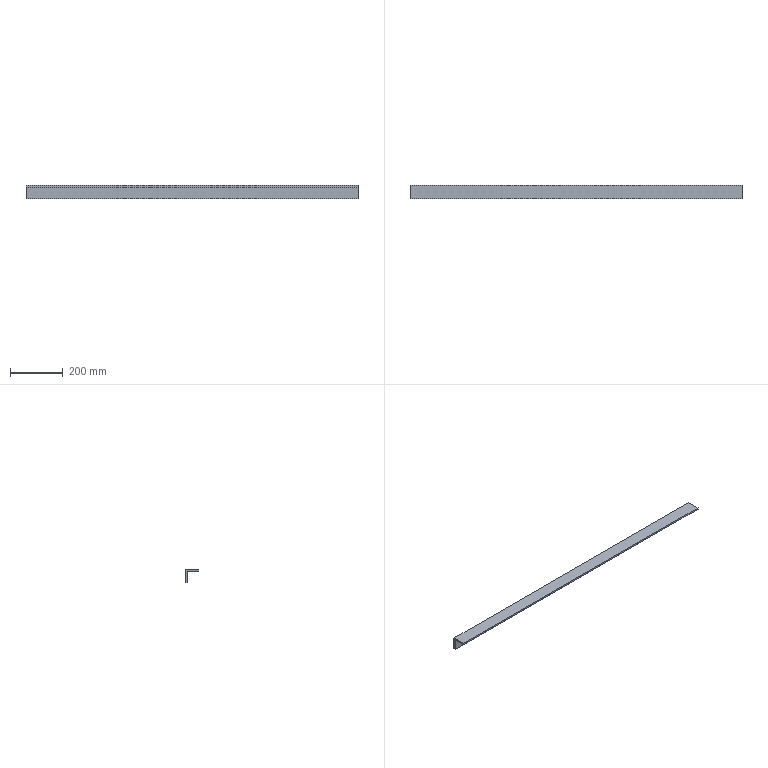Component | NX | LENGTH_CORNER_PROTECTOR_2 | 1 solid | 8 faces | box 1262 x 50 x 50 mm | volume 711768 mm3 | plane 8
STEP:
#1=CARTESIAN_POINT('',(0.,0.,0.));
#2=DIRECTION('',(0.,0.,1.));
#3=DIRECTION('',(1.,0.,0.));
#4=AXIS2_PLACEMENT_3D('',#1,#2,#3);
#5=CARTESIAN_POINT('',(633.5,527.,931.));
#6=VERTEX_POINT('',#5);
#7=CARTESIAN_POINT('',(633.5,527.,981.));
#8=VERTEX_POINT('',#7);
#9=CARTESIAN_POINT('',(633.5,527.,0.));
#10=DIRECTION('',(0.,-0.,1.));
#11=VECTOR('',#10,1.);
#12=LINE('',#9,#11);
#13=CARTESIAN_POINT('',(633.5,-1095.,990.));
#14=DIRECTION('',(-1.,0.,0.));
#15=DIRECTION('',(0.,0.,1.));
#16=AXIS2_PLACEMENT_3D('',#13,#14,#15);
#17=PLANE('',#16);
#18=CARTESIAN_POINT('',(-990.,1622.));
#19=DIRECTION('',(1.,-0.));
#20=VECTOR('',#19,1.);
#21=LINE('',#18,#20);
#22=(GEOMETRIC_REPRESENTATION_CONTEXT(2)PARAMETRIC_REPRESENTATION_CONTEXT()REPRESENTATION_CONTEXT('',''));
#23=DEFINITIONAL_REPRESENTATION('',(#21),#22);
#24=PCURVE('',#17,#23);
#25=CARTESIAN_POINT('',(-628.5,527.,0.));
#26=DIRECTION('',(-0.,1.,0.));
#27=DIRECTION('',(-1.,-0.,0.));
#28=AXIS2_PLACEMENT_3D('',#25,#26,#27);
#29=PLANE('',#28);
#30=CARTESIAN_POINT('',(-1262.,0.));
#31=DIRECTION('',(0.,1.));
#32=VECTOR('',#31,1.);
#33=LINE('',#30,#32);
#34=(GEOMETRIC_REPRESENTATION_CONTEXT(2)PARAMETRIC_REPRESENTATION_CONTEXT()REPRESENTATION_CONTEXT('',''));
#35=DEFINITIONAL_REPRESENTATION('',(#33),#34);
#36=PCURVE('',#29,#35);
#37=SURFACE_CURVE('',#12,(#24,#36),.PCURVE_S1.);
#38=EDGE_CURVE('',#6,#8,#37,.T.);
#39=ORIENTED_EDGE('',*,*,#38,.T.);
#40=CARTESIAN_POINT('',(633.5,477.,981.));
#41=VERTEX_POINT('',#40);
#42=CARTESIAN_POINT('',(633.5,521.,981.));
#43=DIRECTION('',(0.,-1.,0.));
#44=VECTOR('',#43,1.);
#45=LINE('',#42,#44);
#46=CARTESIAN_POINT('',(-9.,1616.));
#47=DIRECTION('',(0.,-1.));
#48=VECTOR('',#47,1.);
#49=LINE('',#46,#48);
#50=(GEOMETRIC_REPRESENTATION_CONTEXT(2)PARAMETRIC_REPRESENTATION_CONTEXT()REPRESENTATION_CONTEXT('',''));
#51=DEFINITIONAL_REPRESENTATION('',(#49),#50);
#52=PCURVE('',#17,#51);
#53=CARTESIAN_POINT('',(-628.5,521.,981.));
#54=DIRECTION('',(0.,0.,1.));
#55=DIRECTION('',(0.7071,0.7071,0.));
#56=AXIS2_PLACEMENT_3D('',#53,#54,#55);
#57=PLANE('',#56);
#58=CARTESIAN_POINT('',(892.369,-892.369));
#59=DIRECTION('',(-0.7071,-0.7071));
#60=VECTOR('',#59,1.);
#61=LINE('',#58,#60);
#62=(GEOMETRIC_REPRESENTATION_CONTEXT(2)PARAMETRIC_REPRESENTATION_CONTEXT()REPRESENTATION_CONTEXT('',''));
#63=DEFINITIONAL_REPRESENTATION('',(#61),#62);
#64=PCURVE('',#57,#63);
#65=SURFACE_CURVE('',#45,(#52,#64),.PCURVE_S1.);
#66=EDGE_CURVE('',#8,#41,#65,.T.);
#67=ORIENTED_EDGE('',*,*,#66,.T.);
#68=CARTESIAN_POINT('',(633.5,477.,975.));
#69=VERTEX_POINT('',#68);
#70=CARTESIAN_POINT('',(633.5,477.,975.));
#71=DIRECTION('',(0.,0.,-1.));
#72=VECTOR('',#71,1.);
#73=LINE('',#70,#72);
#74=CARTESIAN_POINT('',(-15.,1572.));
#75=DIRECTION('',(-1.,0.));
#76=VECTOR('',#75,1.);
#77=LINE('',#74,#76);
#78=(GEOMETRIC_REPRESENTATION_CONTEXT(2)PARAMETRIC_REPRESENTATION_CONTEXT()REPRESENTATION_CONTEXT('',''));
#79=DEFINITIONAL_REPRESENTATION('',(#77),#78);
#80=PCURVE('',#17,#79);
#81=CARTESIAN_POINT('',(-628.5,477.,975.));
#82=DIRECTION('',(0.,-1.,0.));
#83=DIRECTION('',(1.,0.,0.));
#84=AXIS2_PLACEMENT_3D('',#81,#82,#83);
#85=PLANE('',#84);
#86=CARTESIAN_POINT('',(1262.,0.));
#87=DIRECTION('',(0.,-1.));
#88=VECTOR('',#87,1.);
#89=LINE('',#86,#88);
#90=(GEOMETRIC_REPRESENTATION_CONTEXT(2)PARAMETRIC_REPRESENTATION_CONTEXT()REPRESENTATION_CONTEXT('',''));
#91=DEFINITIONAL_REPRESENTATION('',(#89),#90);
#92=PCURVE('',#85,#91);
#93=SURFACE_CURVE('',#73,(#80,#92),.PCURVE_S1.);
#94=EDGE_CURVE('',#41,#69,#93,.T.);
#95=ORIENTED_EDGE('',*,*,#94,.T.);
#96=CARTESIAN_POINT('',(633.5,521.,975.));
#97=VERTEX_POINT('',#96);
#98=CARTESIAN_POINT('',(633.5,521.,975.));
#99=DIRECTION('',(0.,-1.,0.));
#100=VECTOR('',#99,1.);
#101=LINE('',#98,#100);
#102=CARTESIAN_POINT('',(-15.,1616.));
#103=DIRECTION('',(0.,-1.));
#104=VECTOR('',#103,1.);
#105=LINE('',#102,#104);
#106=(GEOMETRIC_REPRESENTATION_CONTEXT(2)PARAMETRIC_REPRESENTATION_CONTEXT()REPRESENTATION_CONTEXT('',''));
#107=DEFINITIONAL_REPRESENTATION('',(#105),#106);
#108=PCURVE('',#17,#107);
#109=CARTESIAN_POINT('',(-628.5,521.,975.));
#110=DIRECTION('',(0.,0.,1.));
#111=DIRECTION('',(0.7071,0.7071,0.));
#112=AXIS2_PLACEMENT_3D('',#109,#110,#111);
#113=PLANE('',#112);
#114=CARTESIAN_POINT('',(892.369,-892.369));
#115=DIRECTION('',(-0.7071,-0.7071));
#116=VECTOR('',#115,1.);
#117=LINE('',#114,#116);
#118=(GEOMETRIC_REPRESENTATION_CONTEXT(2)PARAMETRIC_REPRESENTATION_CONTEXT()REPRESENTATION_CONTEXT('',''));
#119=DEFINITIONAL_REPRESENTATION('',(#117),#118);
#120=PCURVE('',#113,#119);
#121=SURFACE_CURVE('',#101,(#108,#120),.PCURVE_S1.);
#122=EDGE_CURVE('',#97,#69,#121,.T.);
#123=ORIENTED_EDGE('',*,*,#122,.F.);
#124=CARTESIAN_POINT('',(633.5,521.,931.));
#125=VERTEX_POINT('',#124);
#126=CARTESIAN_POINT('',(633.5,521.,0.));
#127=DIRECTION('',(0.,-0.,1.));
#128=VECTOR('',#127,1.);
#129=LINE('',#126,#128);
#130=CARTESIAN_POINT('',(-990.,1616.));
#131=DIRECTION('',(1.,-0.));
#132=VECTOR('',#131,1.);
#133=LINE('',#130,#132);
#134=(GEOMETRIC_REPRESENTATION_CONTEXT(2)PARAMETRIC_REPRESENTATION_CONTEXT()REPRESENTATION_CONTEXT('',''));
#135=DEFINITIONAL_REPRESENTATION('',(#133),#134);
#136=PCURVE('',#17,#135);
#137=CARTESIAN_POINT('',(-628.5,521.,0.));
#138=DIRECTION('',(-0.,1.,0.));
#139=DIRECTION('',(-1.,-0.,0.));
#140=AXIS2_PLACEMENT_3D('',#137,#138,#139);
#141=PLANE('',#140);
#142=CARTESIAN_POINT('',(-1262.,0.));
#143=DIRECTION('',(0.,1.));
#144=VECTOR('',#143,1.);
#145=LINE('',#142,#144);
#146=(GEOMETRIC_REPRESENTATION_CONTEXT(2)PARAMETRIC_REPRESENTATION_CONTEXT()REPRESENTATION_CONTEXT('',''));
#147=DEFINITIONAL_REPRESENTATION('',(#145),#146);
#148=PCURVE('',#141,#147);
#149=SURFACE_CURVE('',#129,(#136,#148),.PCURVE_S1.);
#150=EDGE_CURVE('',#125,#97,#149,.T.);
#151=ORIENTED_EDGE('',*,*,#150,.F.);
#152=CARTESIAN_POINT('',(633.5,521.,931.));
#153=DIRECTION('',(0.,1.,0.));
#154=VECTOR('',#153,1.);
#155=LINE('',#152,#154);
#156=CARTESIAN_POINT('',(-59.,1616.));
#157=DIRECTION('',(0.,1.));
#158=VECTOR('',#157,1.);
#159=LINE('',#156,#158);
#160=(GEOMETRIC_REPRESENTATION_CONTEXT(2)PARAMETRIC_REPRESENTATION_CONTEXT()REPRESENTATION_CONTEXT('',''));
#161=DEFINITIONAL_REPRESENTATION('',(#159),#160);
#162=PCURVE('',#17,#161);
#163=CARTESIAN_POINT('',(-628.5,521.,931.));
#164=DIRECTION('',(0.,-0.,1.));
#165=DIRECTION('',(1.,0.,0.));
#166=AXIS2_PLACEMENT_3D('',#163,#164,#165);
#167=PLANE('',#166);
#168=CARTESIAN_POINT('',(1262.,-0.));
#169=DIRECTION('',(0.,1.));
#170=VECTOR('',#169,1.);
#171=LINE('',#168,#170);
#172=(GEOMETRIC_REPRESENTATION_CONTEXT(2)PARAMETRIC_REPRESENTATION_CONTEXT()REPRESENTATION_CONTEXT('',''));
#173=DEFINITIONAL_REPRESENTATION('',(#171),#172);
#174=PCURVE('',#167,#173);
#175=SURFACE_CURVE('',#155,(#162,#174),.PCURVE_S1.);
#176=EDGE_CURVE('',#125,#6,#175,.T.);
#177=ORIENTED_EDGE('',*,*,#176,.T.);
#178=EDGE_LOOP('',(#39,#67,#95,#123,#151,#177));
#179=FACE_BOUND('',#178,.T.);
#180=ADVANCED_FACE('',(#179),#17,.F.);
#181=ORIENTED_EDGE('',*,*,#176,.F.);
#182=CARTESIAN_POINT('',(-628.5,521.,931.));
#183=VERTEX_POINT('',#182);
#184=CARTESIAN_POINT('',(-628.5,521.,931.));
#185=DIRECTION('',(1.,0.,0.));
#186=VECTOR('',#185,1.);
#187=LINE('',#184,#186);
#188=CARTESIAN_POINT('',(0.,0.));
#189=DIRECTION('',(1.,0.));
#190=VECTOR('',#189,1.);
#191=LINE('',#188,#190);
#192=(GEOMETRIC_REPRESENTATION_CONTEXT(2)PARAMETRIC_REPRESENTATION_CONTEXT()REPRESENTATION_CONTEXT('',''));
#193=DEFINITIONAL_REPRESENTATION('',(#191),#192);
#194=PCURVE('',#167,#193);
#195=CARTESIAN_POINT('',(0.,931.));
#196=DIRECTION('',(-1.,0.));
#197=VECTOR('',#196,1.);
#198=LINE('',#195,#197);
#199=(GEOMETRIC_REPRESENTATION_CONTEXT(2)PARAMETRIC_REPRESENTATION_CONTEXT()REPRESENTATION_CONTEXT('',''));
#200=DEFINITIONAL_REPRESENTATION('',(#198),#199);
#201=PCURVE('',#141,#200);
#202=SURFACE_CURVE('',#187,(#194,#201),.PCURVE_S1.);
#203=EDGE_CURVE('',#183,#125,#202,.T.);
#204=ORIENTED_EDGE('',*,*,#203,.F.);
#205=CARTESIAN_POINT('',(-628.5,527.,931.));
#206=VERTEX_POINT('',#205);
#207=CARTESIAN_POINT('',(-628.5,521.,931.));
#208=DIRECTION('',(-0.,1.,0.));
#209=VECTOR('',#208,1.);
#210=LINE('',#207,#209);
#211=CARTESIAN_POINT('',(0.,0.));
#212=DIRECTION('',(0.,1.));
#213=VECTOR('',#212,1.);
#214=LINE('',#211,#213);
#215=(GEOMETRIC_REPRESENTATION_CONTEXT(2)PARAMETRIC_REPRESENTATION_CONTEXT()REPRESENTATION_CONTEXT('',''));
#216=DEFINITIONAL_REPRESENTATION('',(#214),#215);
#217=PCURVE('',#167,#216);
#218=CARTESIAN_POINT('',(-628.5,521.,975.));
#219=DIRECTION('',(-1.,-0.,0.));
#220=DIRECTION('',(0.,-1.,0.));
#221=AXIS2_PLACEMENT_3D('',#218,#219,#220);
#222=PLANE('',#221);
#223=CARTESIAN_POINT('',(0.,-44.));
#224=DIRECTION('',(-1.,0.));
#225=VECTOR('',#224,1.);
#226=LINE('',#223,#225);
#227=(GEOMETRIC_REPRESENTATION_CONTEXT(2)PARAMETRIC_REPRESENTATION_CONTEXT()REPRESENTATION_CONTEXT('',''));
#228=DEFINITIONAL_REPRESENTATION('',(#226),#227);
#229=PCURVE('',#222,#228);
#230=SURFACE_CURVE('',#210,(#217,#229),.PCURVE_S1.);
#231=EDGE_CURVE('',#183,#206,#230,.T.);
#232=ORIENTED_EDGE('',*,*,#231,.T.);
#233=CARTESIAN_POINT('',(-628.5,527.,931.));
#234=DIRECTION('',(1.,0.,0.));
#235=VECTOR('',#234,1.);
#236=LINE('',#233,#235);
#237=CARTESIAN_POINT('',(0.,6.));
#238=DIRECTION('',(1.,0.));
#239=VECTOR('',#238,1.);
#240=LINE('',#237,#239);
#241=(GEOMETRIC_REPRESENTATION_CONTEXT(2)PARAMETRIC_REPRESENTATION_CONTEXT()REPRESENTATION_CONTEXT('',''));
#242=DEFINITIONAL_REPRESENTATION('',(#240),#241);
#243=PCURVE('',#167,#242);
#244=CARTESIAN_POINT('',(0.,931.));
#245=DIRECTION('',(-1.,0.));
#246=VECTOR('',#245,1.);
#247=LINE('',#244,#246);
#248=(GEOMETRIC_REPRESENTATION_CONTEXT(2)PARAMETRIC_REPRESENTATION_CONTEXT()REPRESENTATION_CONTEXT('',''));
#249=DEFINITIONAL_REPRESENTATION('',(#247),#248);
#250=PCURVE('',#29,#249);
#251=SURFACE_CURVE('',#236,(#243,#250),.PCURVE_S1.);
#252=EDGE_CURVE('',#206,#6,#251,.T.);
#253=ORIENTED_EDGE('',*,*,#252,.T.);
#254=EDGE_LOOP('',(#181,#204,#232,#253));
#255=FACE_BOUND('',#254,.T.);
#256=ADVANCED_FACE('',(#255),#167,.F.);
#257=CARTESIAN_POINT('',(-628.5,527.,981.));
#258=VERTEX_POINT('',#257);
#259=CARTESIAN_POINT('',(-628.5,477.,981.));
#260=VERTEX_POINT('',#259);
#261=CARTESIAN_POINT('',(-628.5,521.,981.));
#262=DIRECTION('',(0.,-1.,0.));
#263=VECTOR('',#262,1.);
#264=LINE('',#261,#263);
#265=CARTESIAN_POINT('',(0.,6.));
#266=DIRECTION('',(1.,0.));
#267=VECTOR('',#266,1.);
#268=LINE('',#265,#267);
#269=(GEOMETRIC_REPRESENTATION_CONTEXT(2)PARAMETRIC_REPRESENTATION_CONTEXT()REPRESENTATION_CONTEXT('',''));
#270=DEFINITIONAL_REPRESENTATION('',(#268),#269);
#271=PCURVE('',#222,#270);
#272=CARTESIAN_POINT('',(0.,0.));
#273=DIRECTION('',(-0.7071,-0.7071));
#274=VECTOR('',#273,1.);
#275=LINE('',#272,#274);
#276=(GEOMETRIC_REPRESENTATION_CONTEXT(2)PARAMETRIC_REPRESENTATION_CONTEXT()REPRESENTATION_CONTEXT('',''));
#277=DEFINITIONAL_REPRESENTATION('',(#275),#276);
#278=PCURVE('',#57,#277);
#279=SURFACE_CURVE('',#264,(#271,#278),.PCURVE_S1.);
#280=EDGE_CURVE('',#258,#260,#279,.T.);
#281=ORIENTED_EDGE('',*,*,#280,.F.);
#282=CARTESIAN_POINT('',(-628.5,527.,0.));
#283=DIRECTION('',(0.,-0.,1.));
#284=VECTOR('',#283,1.);
#285=LINE('',#282,#284);
#286=CARTESIAN_POINT('',(-6.,-975.));
#287=DIRECTION('',(0.,1.));
#288=VECTOR('',#287,1.);
#289=LINE('',#286,#288);
#290=(GEOMETRIC_REPRESENTATION_CONTEXT(2)PARAMETRIC_REPRESENTATION_CONTEXT()REPRESENTATION_CONTEXT('',''));
#291=DEFINITIONAL_REPRESENTATION('',(#289),#290);
#292=PCURVE('',#222,#291);
#293=CARTESIAN_POINT('',(0.,0.));
#294=DIRECTION('',(0.,1.));
#295=VECTOR('',#294,1.);
#296=LINE('',#293,#295);
#297=(GEOMETRIC_REPRESENTATION_CONTEXT(2)PARAMETRIC_REPRESENTATION_CONTEXT()REPRESENTATION_CONTEXT('',''));
#298=DEFINITIONAL_REPRESENTATION('',(#296),#297);
#299=PCURVE('',#29,#298);
#300=SURFACE_CURVE('',#285,(#292,#299),.PCURVE_S1.);
#301=EDGE_CURVE('',#206,#258,#300,.T.);
#302=ORIENTED_EDGE('',*,*,#301,.F.);
#303=ORIENTED_EDGE('',*,*,#231,.F.);
#304=CARTESIAN_POINT('',(-628.5,521.,975.));
#305=VERTEX_POINT('',#304);
#306=CARTESIAN_POINT('',(-628.5,521.,0.));
#307=DIRECTION('',(-0.,-0.,1.));
#308=VECTOR('',#307,1.);
#309=LINE('',#306,#308);
#310=CARTESIAN_POINT('',(0.,-975.));
#311=DIRECTION('',(0.,1.));
#312=VECTOR('',#311,1.);
#313=LINE('',#310,#312);
#314=(GEOMETRIC_REPRESENTATION_CONTEXT(2)PARAMETRIC_REPRESENTATION_CONTEXT()REPRESENTATION_CONTEXT('',''));
#315=DEFINITIONAL_REPRESENTATION('',(#313),#314);
#316=PCURVE('',#222,#315);
#317=CARTESIAN_POINT('',(0.,0.));
#318=DIRECTION('',(0.,1.));
#319=VECTOR('',#318,1.);
#320=LINE('',#317,#319);
#321=(GEOMETRIC_REPRESENTATION_CONTEXT(2)PARAMETRIC_REPRESENTATION_CONTEXT()REPRESENTATION_CONTEXT('',''));
#322=DEFINITIONAL_REPRESENTATION('',(#320),#321);
#323=PCURVE('',#141,#322);
#324=SURFACE_CURVE('',#309,(#316,#323),.PCURVE_S1.);
#325=EDGE_CURVE('',#183,#305,#324,.T.);
#326=ORIENTED_EDGE('',*,*,#325,.T.);
#327=CARTESIAN_POINT('',(-628.5,477.,975.));
#328=VERTEX_POINT('',#327);
#329=CARTESIAN_POINT('',(-628.5,521.,975.));
#330=DIRECTION('',(0.,-1.,0.));
#331=VECTOR('',#330,1.);
#332=LINE('',#329,#331);
#333=CARTESIAN_POINT('',(0.,0.));
#334=DIRECTION('',(1.,0.));
#335=VECTOR('',#334,1.);
#336=LINE('',#333,#335);
#337=(GEOMETRIC_REPRESENTATION_CONTEXT(2)PARAMETRIC_REPRESENTATION_CONTEXT()REPRESENTATION_CONTEXT('',''));
#338=DEFINITIONAL_REPRESENTATION('',(#336),#337);
#339=PCURVE('',#222,#338);
#340=CARTESIAN_POINT('',(0.,0.));
#341=DIRECTION('',(-0.7071,-0.7071));
#342=VECTOR('',#341,1.);
#343=LINE('',#340,#342);
#344=(GEOMETRIC_REPRESENTATION_CONTEXT(2)PARAMETRIC_REPRESENTATION_CONTEXT()REPRESENTATION_CONTEXT('',''));
#345=DEFINITIONAL_REPRESENTATION('',(#343),#344);
#346=PCURVE('',#113,#345);
#347=SURFACE_CURVE('',#332,(#339,#346),.PCURVE_S1.);
#348=EDGE_CURVE('',#305,#328,#347,.T.);
#349=ORIENTED_EDGE('',*,*,#348,.T.);
#350=CARTESIAN_POINT('',(-628.5,477.,975.));
#351=DIRECTION('',(0.,0.,1.));
#352=VECTOR('',#351,1.);
#353=LINE('',#350,#352);
#354=CARTESIAN_POINT('',(44.,0.));
#355=DIRECTION('',(0.,1.));
#356=VECTOR('',#355,1.);
#357=LINE('',#354,#356);
#358=(GEOMETRIC_REPRESENTATION_CONTEXT(2)PARAMETRIC_REPRESENTATION_CONTEXT()REPRESENTATION_CONTEXT('',''));
#359=DEFINITIONAL_REPRESENTATION('',(#357),#358);
#360=PCURVE('',#222,#359);
#361=CARTESIAN_POINT('',(0.,0.));
#362=DIRECTION('',(0.,1.));
#363=VECTOR('',#362,1.);
#364=LINE('',#361,#363);
#365=(GEOMETRIC_REPRESENTATION_CONTEXT(2)PARAMETRIC_REPRESENTATION_CONTEXT()REPRESENTATION_CONTEXT('',''));
#366=DEFINITIONAL_REPRESENTATION('',(#364),#365);
#367=PCURVE('',#85,#366);
#368=SURFACE_CURVE('',#353,(#360,#367),.PCURVE_S1.);
#369=EDGE_CURVE('',#328,#260,#368,.T.);
#370=ORIENTED_EDGE('',*,*,#369,.T.);
#371=EDGE_LOOP('',(#281,#302,#303,#326,#349,#370));
#372=FACE_BOUND('',#371,.T.);
#373=ADVANCED_FACE('',(#372),#222,.T.);
#374=ORIENTED_EDGE('',*,*,#94,.F.);
#375=CARTESIAN_POINT('',(-628.5,477.,981.));
#376=DIRECTION('',(1.,0.,0.));
#377=VECTOR('',#376,1.);
#378=LINE('',#375,#377);
#379=CARTESIAN_POINT('',(0.,6.));
#380=DIRECTION('',(1.,0.));
#381=VECTOR('',#380,1.);
#382=LINE('',#379,#381);
#383=(GEOMETRIC_REPRESENTATION_CONTEXT(2)PARAMETRIC_REPRESENTATION_CONTEXT()REPRESENTATION_CONTEXT('',''));
#384=DEFINITIONAL_REPRESENTATION('',(#382),#383);
#385=PCURVE('',#85,#384);
#386=CARTESIAN_POINT('',(-31.113,-31.113));
#387=DIRECTION('',(0.7071,-0.7071));
#388=VECTOR('',#387,1.);
#389=LINE('',#386,#388);
#390=(GEOMETRIC_REPRESENTATION_CONTEXT(2)PARAMETRIC_REPRESENTATION_CONTEXT()REPRESENTATION_CONTEXT('',''));
#391=DEFINITIONAL_REPRESENTATION('',(#389),#390);
#392=PCURVE('',#57,#391);
#393=SURFACE_CURVE('',#378,(#385,#392),.PCURVE_S1.);
#394=EDGE_CURVE('',#260,#41,#393,.T.);
#395=ORIENTED_EDGE('',*,*,#394,.F.);
#396=ORIENTED_EDGE('',*,*,#369,.F.);
#397=CARTESIAN_POINT('',(-628.5,477.,975.));
#398=DIRECTION('',(1.,0.,0.));
#399=VECTOR('',#398,1.);
#400=LINE('',#397,#399);
#401=CARTESIAN_POINT('',(0.,0.));
#402=DIRECTION('',(1.,0.));
#403=VECTOR('',#402,1.);
#404=LINE('',#401,#403);
#405=(GEOMETRIC_REPRESENTATION_CONTEXT(2)PARAMETRIC_REPRESENTATION_CONTEXT()REPRESENTATION_CONTEXT('',''));
#406=DEFINITIONAL_REPRESENTATION('',(#404),#405);
#407=PCURVE('',#85,#406);
#408=CARTESIAN_POINT('',(-31.113,-31.113));
#409=DIRECTION('',(0.7071,-0.7071));
#410=VECTOR('',#409,1.);
#411=LINE('',#408,#410);
#412=(GEOMETRIC_REPRESENTATION_CONTEXT(2)PARAMETRIC_REPRESENTATION_CONTEXT()REPRESENTATION_CONTEXT('',''));
#413=DEFINITIONAL_REPRESENTATION('',(#411),#412);
#414=PCURVE('',#113,#413);
#415=SURFACE_CURVE('',#400,(#407,#414),.PCURVE_S1.);
#416=EDGE_CURVE('',#328,#69,#415,.T.);
#417=ORIENTED_EDGE('',*,*,#416,.T.);
#418=EDGE_LOOP('',(#374,#395,#396,#417));
#419=FACE_BOUND('',#418,.T.);
#420=ADVANCED_FACE('',(#419),#85,.T.);
#421=ORIENTED_EDGE('',*,*,#203,.T.);
#422=ORIENTED_EDGE('',*,*,#150,.T.);
#423=CARTESIAN_POINT('',(-628.5,521.,975.));
#424=DIRECTION('',(1.,0.,0.));
#425=VECTOR('',#424,1.);
#426=LINE('',#423,#425);
#427=CARTESIAN_POINT('',(0.,975.));
#428=DIRECTION('',(-1.,0.));
#429=VECTOR('',#428,1.);
#430=LINE('',#427,#429);
#431=(GEOMETRIC_REPRESENTATION_CONTEXT(2)PARAMETRIC_REPRESENTATION_CONTEXT()REPRESENTATION_CONTEXT('',''));
#432=DEFINITIONAL_REPRESENTATION('',(#430),#431);
#433=PCURVE('',#141,#432);
#434=CARTESIAN_POINT('',(0.,0.));
#435=DIRECTION('',(0.7071,-0.7071));
#436=VECTOR('',#435,1.);
#437=LINE('',#434,#436);
#438=(GEOMETRIC_REPRESENTATION_CONTEXT(2)PARAMETRIC_REPRESENTATION_CONTEXT()REPRESENTATION_CONTEXT('',''));
#439=DEFINITIONAL_REPRESENTATION('',(#437),#438);
#440=PCURVE('',#113,#439);
#441=SURFACE_CURVE('',#426,(#433,#440),.PCURVE_S1.);
#442=EDGE_CURVE('',#305,#97,#441,.T.);
#443=ORIENTED_EDGE('',*,*,#442,.F.);
#444=ORIENTED_EDGE('',*,*,#325,.F.);
#445=EDGE_LOOP('',(#421,#422,#443,#444));
#446=FACE_BOUND('',#445,.T.);
#447=ADVANCED_FACE('',(#446),#141,.F.);
#448=ORIENTED_EDGE('',*,*,#442,.T.);
#449=ORIENTED_EDGE('',*,*,#122,.T.);
#450=ORIENTED_EDGE('',*,*,#416,.F.);
#451=ORIENTED_EDGE('',*,*,#348,.F.);
#452=EDGE_LOOP('',(#448,#449,#450,#451));
#453=FACE_BOUND('',#452,.T.);
#454=ADVANCED_FACE('',(#453),#113,.F.);
#455=ORIENTED_EDGE('',*,*,#38,.F.);
#456=ORIENTED_EDGE('',*,*,#252,.F.);
#457=ORIENTED_EDGE('',*,*,#301,.T.);
#458=CARTESIAN_POINT('',(-628.5,527.,981.));
#459=DIRECTION('',(1.,0.,0.));
#460=VECTOR('',#459,1.);
#461=LINE('',#458,#460);
#462=CARTESIAN_POINT('',(0.,981.));
#463=DIRECTION('',(-1.,0.));
#464=VECTOR('',#463,1.);
#465=LINE('',#462,#464);
#466=(GEOMETRIC_REPRESENTATION_CONTEXT(2)PARAMETRIC_REPRESENTATION_CONTEXT()REPRESENTATION_CONTEXT('',''));
#467=DEFINITIONAL_REPRESENTATION('',(#465),#466);
#468=PCURVE('',#29,#467);
#469=CARTESIAN_POINT('',(4.243,4.243));
#470=DIRECTION('',(0.7071,-0.7071));
#471=VECTOR('',#470,1.);
#472=LINE('',#469,#471);
#473=(GEOMETRIC_REPRESENTATION_CONTEXT(2)PARAMETRIC_REPRESENTATION_CONTEXT()REPRESENTATION_CONTEXT('',''));
#474=DEFINITIONAL_REPRESENTATION('',(#472),#473);
#475=PCURVE('',#57,#474);
#476=SURFACE_CURVE('',#461,(#468,#475),.PCURVE_S1.);
#477=EDGE_CURVE('',#258,#8,#476,.T.);
#478=ORIENTED_EDGE('',*,*,#477,.T.);
#479=EDGE_LOOP('',(#455,#456,#457,#478));
#480=FACE_BOUND('',#479,.T.);
#481=ADVANCED_FACE('',(#480),#29,.T.);
#482=ORIENTED_EDGE('',*,*,#66,.F.);
#483=ORIENTED_EDGE('',*,*,#477,.F.);
#484=ORIENTED_EDGE('',*,*,#280,.T.);
#485=ORIENTED_EDGE('',*,*,#394,.T.);
#486=EDGE_LOOP('',(#482,#483,#484,#485));
#487=FACE_BOUND('',#486,.T.);
#488=ADVANCED_FACE('',(#487),#57,.T.);
#489=CLOSED_SHELL('',(#180,#256,#373,#420,#447,#454,#481,#488));
#490=MANIFOLD_SOLID_BREP('',#489);
#491=(LENGTH_UNIT()NAMED_UNIT(*)SI_UNIT(.MILLI.,.METRE.));
#492=UNCERTAINTY_MEASURE_WITH_UNIT(LENGTH_MEASURE(0.0000001),#491,'','');
#493=(NAMED_UNIT(*)PLANE_ANGLE_UNIT()SI_UNIT($,.RADIAN.));
#494=(NAMED_UNIT(*)SI_UNIT($,.STERADIAN.)SOLID_ANGLE_UNIT());
#495=(GEOMETRIC_REPRESENTATION_CONTEXT(3)GLOBAL_UNCERTAINTY_ASSIGNED_CONTEXT((#492))GLOBAL_UNIT_ASSIGNED_CONTEXT((#491,#493,#494))REPRESENTATION_CONTEXT('',''));
#496=ADVANCED_BREP_SHAPE_REPRESENTATION('',(#4,#490),#495);